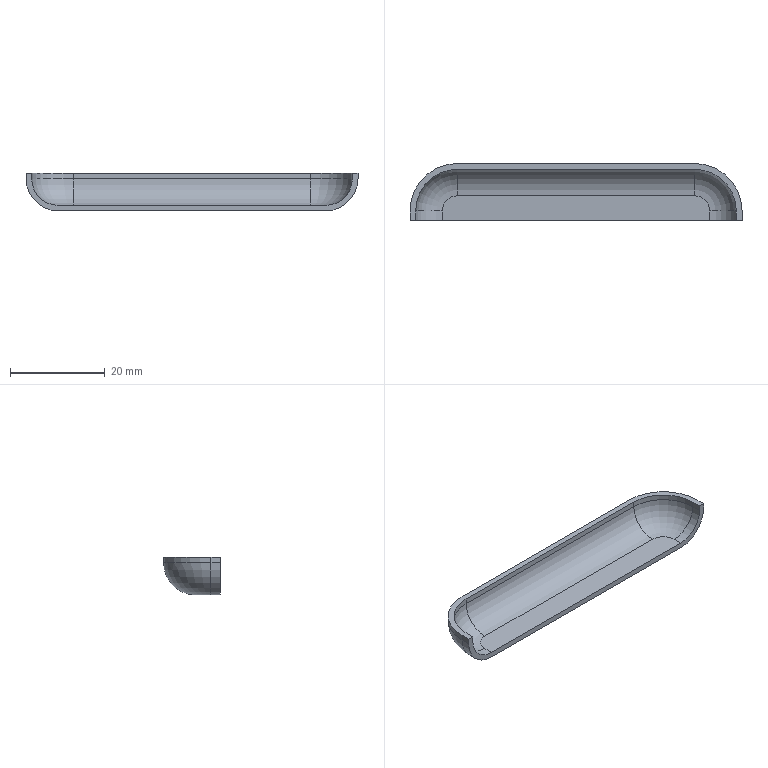Component | SolidWorks | LeftDoorPanelAssembly-1_LeftDoorPanelWeldment-1_LouverSupplement-12 | 1 solid | 24 faces | box 70 x 12 x 8 mm | volume 1361 mm3 | cylinder 10 | plane 10 | torus 4 | commonest cylinder face diameters 13.6 x3 11.2 x3 20 x2 17.6 x2
build123d program:
from build123d import *

# Parameters (mm, degrees)
BOSS_EXTRUDE1_DEPTH = 8
FILLET1_R           = 6.8
SHELL1_T            = -1.2


with BuildPart() as part:
    # Sketch1 → Boss-Extrude1 (new body)
    with BuildSketch(Plane.XY):
        with BuildLine():
            Line((-25, 12), (25, 12))
            ThreePointArc((25, 12), (32.071, 9.071), (35, 2))
            Line((35, 2), (35, 0))
            Line((35, 0), (-35, 0))
            Line((-35, 0), (-35, 2))
            ThreePointArc((-35, 2), (-32.071, 9.071), (-25, 12))
        make_face()
    extrude(amount=BOSS_EXTRUDE1_DEPTH)

    # Fillet1
    fillet1_edges = [part.edges().sort_by_distance(p)[0] for p in [
        (35, 1, 8),
        (32.071, 9.071, 8),
        (0, 12, 8),
        (-32.071, 9.071, 8),
        (-35, 1, 8),
    ]]
    fillet(fillet1_edges, radius=FILLET1_R)

    # Shell1
    shell1_openings = [part.faces().sort_by_distance(p)[0] for p in [
        (0, 0, 3.909),
        (0, 5.797, 0),
    ]]
    offset(amount=SHELL1_T, openings=shell1_openings, kind=Kind.INTERSECTION)


solid = part.part

# Placed as in the assembly
solid = solid.moved(Location((224.337, 24.042, -71.9), (-180, 0, 180)))
STEP:
#1=COLOUR_RGB('',0.7922,0.8196,0.9333);
#2=FILL_AREA_STYLE_COLOUR('',#1);
#3=FILL_AREA_STYLE('',(#2));
#4=SURFACE_STYLE_FILL_AREA(#3);
#5=SURFACE_SIDE_STYLE('',(#4));
#6=SURFACE_STYLE_USAGE(.BOTH.,#5);
#7=PRESENTATION_STYLE_ASSIGNMENT((#6));
#8=CARTESIAN_POINT('',(10.21,1.025,-2.878));
#9=VERTEX_POINT('',#8);
#10=CARTESIAN_POINT('',(10.21,1.025,-2.831));
#11=VERTEX_POINT('',#10);
#12=CARTESIAN_POINT('',(10.21,1.025,-3.146));
#13=DIRECTION('',(-0.,0.,1.));
#14=VECTOR('',#13,39.37);
#15=LINE('',#12,#14);
#16=EDGE_CURVE('',#9,#11,#15,.T.);
#17=ORIENTED_EDGE('',*,*,#16,.F.);
#18=CARTESIAN_POINT('',(9.816,1.419,-2.878));
#19=VERTEX_POINT('',#18);
#20=CARTESIAN_POINT('',(9.816,1.025,-2.878));
#21=DIRECTION('',(-0.,0.,1.));
#22=DIRECTION('',(-1.,-0.,-0.));
#23=AXIS2_PLACEMENT_3D('',#20,#21,#22);
#24=CIRCLE('',#23,0.3937);
#25=EDGE_CURVE('',#9,#19,#24,.T.);
#26=ORIENTED_EDGE('',*,*,#25,.T.);
#27=CARTESIAN_POINT('',(9.816,1.419,-2.831));
#28=VERTEX_POINT('',#27);
#29=CARTESIAN_POINT('',(9.816,1.419,-3.146));
#30=DIRECTION('',(-0.,0.,1.));
#31=VECTOR('',#30,39.37);
#32=LINE('',#29,#31);
#33=EDGE_CURVE('',#19,#28,#32,.T.);
#34=ORIENTED_EDGE('',*,*,#33,.T.);
#35=CARTESIAN_POINT('',(9.816,1.025,-2.831));
#36=DIRECTION('',(0.,-0.,-1.));
#37=DIRECTION('',(-1.,-0.,-0.));
#38=AXIS2_PLACEMENT_3D('',#35,#36,#37);
#39=CIRCLE('',#38,0.3937);
#40=EDGE_CURVE('',#28,#11,#39,.T.);
#41=ORIENTED_EDGE('',*,*,#40,.T.);
#42=EDGE_LOOP('',(#17,#26,#34,#41));
#43=FACE_OUTER_BOUND('',#42,.T.);
#44=CARTESIAN_POINT('',(9.816,1.025,-3.146));
#45=DIRECTION('',(-0.,0.,1.));
#46=DIRECTION('',(1.,0.,0.));
#47=AXIS2_PLACEMENT_3D('',#44,#45,#46);
#48=CYLINDRICAL_SURFACE('',#47,0.3937);
#49=ADVANCED_FACE('',(#43),#48,.T.);
#50=CARTESIAN_POINT('',(10.21,0.9465,-2.878));
#51=VERTEX_POINT('',#50);
#52=CARTESIAN_POINT('',(10.21,0.9465,-2.831));
#53=VERTEX_POINT('',#52);
#54=CARTESIAN_POINT('',(10.21,0.9465,-3.146));
#55=DIRECTION('',(-0.,0.,1.));
#56=VECTOR('',#55,39.37);
#57=LINE('',#54,#56);
#58=EDGE_CURVE('',#51,#53,#57,.T.);
#59=ORIENTED_EDGE('',*,*,#58,.F.);
#60=CARTESIAN_POINT('',(10.21,1.025,-2.878));
#61=DIRECTION('',(-0.,1.,-0.));
#62=VECTOR('',#61,39.37);
#63=LINE('',#60,#62);
#64=EDGE_CURVE('',#51,#9,#63,.T.);
#65=ORIENTED_EDGE('',*,*,#64,.T.);
#66=ORIENTED_EDGE('',*,*,#16,.T.);
#67=CARTESIAN_POINT('',(10.21,0.9465,-2.831));
#68=DIRECTION('',(0.,-1.,0.));
#69=VECTOR('',#68,39.37);
#70=LINE('',#67,#69);
#71=EDGE_CURVE('',#11,#53,#70,.T.);
#72=ORIENTED_EDGE('',*,*,#71,.T.);
#73=EDGE_LOOP('',(#59,#65,#66,#72));
#74=FACE_OUTER_BOUND('',#73,.T.);
#75=CARTESIAN_POINT('',(10.21,0.9465,-3.146));
#76=DIRECTION('',(-1.,-0.,-0.));
#77=DIRECTION('',(-0.,0.,1.));
#78=AXIS2_PLACEMENT_3D('',#75,#76,#77);
#79=PLANE('',#78);
#80=ADVANCED_FACE('',(#74),#79,.F.);
#81=CARTESIAN_POINT('',(7.501,0.9465,-2.878));
#82=VERTEX_POINT('',#81);
#83=CARTESIAN_POINT('',(7.722,0.9465,-3.098));
#84=VERTEX_POINT('',#83);
#85=CARTESIAN_POINT('',(7.722,0.9465,-2.878));
#86=DIRECTION('',(0.,-1.,0.));
#87=DIRECTION('',(0.,-0.,-1.));
#88=AXIS2_PLACEMENT_3D('',#85,#86,#87);
#89=CIRCLE('',#88,0.2205);
#90=EDGE_CURVE('',#82,#84,#89,.T.);
#91=ORIENTED_EDGE('',*,*,#90,.F.);
#92=CARTESIAN_POINT('',(7.501,0.9465,-2.831));
#93=VERTEX_POINT('',#92);
#94=CARTESIAN_POINT('',(7.501,0.9465,-3.146));
#95=DIRECTION('',(-0.,0.,1.));
#96=VECTOR('',#95,39.37);
#97=LINE('',#94,#96);
#98=EDGE_CURVE('',#82,#93,#97,.T.);
#99=ORIENTED_EDGE('',*,*,#98,.T.);
#100=CARTESIAN_POINT('',(7.454,0.9465,-2.831));
#101=VERTEX_POINT('',#100);
#102=CARTESIAN_POINT('',(10.21,0.9465,-2.831));
#103=DIRECTION('',(-1.,-0.,-0.));
#104=VECTOR('',#103,39.37);
#105=LINE('',#102,#104);
#106=EDGE_CURVE('',#93,#101,#105,.T.);
#107=ORIENTED_EDGE('',*,*,#106,.T.);
#108=CARTESIAN_POINT('',(7.454,0.9465,-2.878));
#109=VERTEX_POINT('',#108);
#110=CARTESIAN_POINT('',(7.454,0.9465,-3.146));
#111=DIRECTION('',(-0.,0.,1.));
#112=VECTOR('',#111,39.37);
#113=LINE('',#110,#112);
#114=EDGE_CURVE('',#109,#101,#113,.T.);
#115=ORIENTED_EDGE('',*,*,#114,.F.);
#116=CARTESIAN_POINT('',(7.722,0.9465,-3.146));
#117=VERTEX_POINT('',#116);
#118=CARTESIAN_POINT('',(7.722,0.9465,-2.878));
#119=DIRECTION('',(0.,-1.,0.));
#120=DIRECTION('',(0.,-0.,-1.));
#121=AXIS2_PLACEMENT_3D('',#118,#119,#120);
#122=CIRCLE('',#121,0.2677);
#123=EDGE_CURVE('',#109,#117,#122,.T.);
#124=ORIENTED_EDGE('',*,*,#123,.T.);
#125=CARTESIAN_POINT('',(9.942,0.9465,-3.146));
#126=VERTEX_POINT('',#125);
#127=CARTESIAN_POINT('',(10.21,0.9465,-3.146));
#128=DIRECTION('',(-1.,-0.,-0.));
#129=VECTOR('',#128,39.37);
#130=LINE('',#127,#129);
#131=EDGE_CURVE('',#126,#117,#130,.T.);
#132=ORIENTED_EDGE('',*,*,#131,.F.);
#133=CARTESIAN_POINT('',(9.942,0.9465,-2.878));
#134=DIRECTION('',(0.,-1.,0.));
#135=DIRECTION('',(0.,-0.,-1.));
#136=AXIS2_PLACEMENT_3D('',#133,#134,#135);
#137=CIRCLE('',#136,0.2677);
#138=EDGE_CURVE('',#126,#51,#137,.T.);
#139=ORIENTED_EDGE('',*,*,#138,.T.);
#140=ORIENTED_EDGE('',*,*,#58,.T.);
#141=CARTESIAN_POINT('',(10.163,0.9465,-2.831));
#142=VERTEX_POINT('',#141);
#143=CARTESIAN_POINT('',(10.21,0.9465,-2.831));
#144=DIRECTION('',(-1.,-0.,-0.));
#145=VECTOR('',#144,39.37);
#146=LINE('',#143,#145);
#147=EDGE_CURVE('',#53,#142,#146,.T.);
#148=ORIENTED_EDGE('',*,*,#147,.T.);
#149=CARTESIAN_POINT('',(10.163,0.9465,-2.878));
#150=VERTEX_POINT('',#149);
#151=CARTESIAN_POINT('',(10.163,0.9465,-3.146));
#152=DIRECTION('',(-0.,0.,1.));
#153=VECTOR('',#152,39.37);
#154=LINE('',#151,#153);
#155=EDGE_CURVE('',#150,#142,#154,.T.);
#156=ORIENTED_EDGE('',*,*,#155,.F.);
#157=CARTESIAN_POINT('',(9.942,0.9465,-3.098));
#158=VERTEX_POINT('',#157);
#159=CARTESIAN_POINT('',(9.942,0.9465,-2.878));
#160=DIRECTION('',(0.,-1.,0.));
#161=DIRECTION('',(0.,-0.,-1.));
#162=AXIS2_PLACEMENT_3D('',#159,#160,#161);
#163=CIRCLE('',#162,0.2205);
#164=EDGE_CURVE('',#158,#150,#163,.T.);
#165=ORIENTED_EDGE('',*,*,#164,.F.);
#166=CARTESIAN_POINT('',(10.21,0.9465,-3.098));
#167=DIRECTION('',(-1.,-0.,-0.));
#168=VECTOR('',#167,39.37);
#169=LINE('',#166,#168);
#170=EDGE_CURVE('',#158,#84,#169,.T.);
#171=ORIENTED_EDGE('',*,*,#170,.T.);
#172=EDGE_LOOP('',(#91,#99,#107,#115,#124,#132,#139,#140,#148,#156,#165,#171));
#173=FACE_OUTER_BOUND('',#172,.T.);
#174=CARTESIAN_POINT('',(10.21,0.9465,-3.146));
#175=DIRECTION('',(-0.,1.,-0.));
#176=DIRECTION('',(0.,-0.,-1.));
#177=AXIS2_PLACEMENT_3D('',#174,#175,#176);
#178=PLANE('',#177);
#179=ADVANCED_FACE('',(#173),#178,.F.);
#180=CARTESIAN_POINT('',(7.454,1.025,-2.878));
#181=VERTEX_POINT('',#180);
#182=CARTESIAN_POINT('',(7.454,1.025,-2.831));
#183=VERTEX_POINT('',#182);
#184=CARTESIAN_POINT('',(7.454,1.025,-3.146));
#185=DIRECTION('',(-0.,0.,1.));
#186=VECTOR('',#185,39.37);
#187=LINE('',#184,#186);
#188=EDGE_CURVE('',#181,#183,#187,.T.);
#189=ORIENTED_EDGE('',*,*,#188,.F.);
#190=CARTESIAN_POINT('',(7.454,0.9465,-2.878));
#191=DIRECTION('',(0.,-1.,0.));
#192=VECTOR('',#191,39.37);
#193=LINE('',#190,#192);
#194=EDGE_CURVE('',#181,#109,#193,.T.);
#195=ORIENTED_EDGE('',*,*,#194,.T.);
#196=ORIENTED_EDGE('',*,*,#114,.T.);
#197=CARTESIAN_POINT('',(7.454,0.9465,-2.831));
#198=DIRECTION('',(-0.,1.,-0.));
#199=VECTOR('',#198,39.37);
#200=LINE('',#197,#199);
#201=EDGE_CURVE('',#101,#183,#200,.T.);
#202=ORIENTED_EDGE('',*,*,#201,.T.);
#203=EDGE_LOOP('',(#189,#195,#196,#202));
#204=FACE_OUTER_BOUND('',#203,.T.);
#205=CARTESIAN_POINT('',(7.454,0.9465,-3.146));
#206=DIRECTION('',(1.,0.,0.));
#207=DIRECTION('',(0.,-0.,-1.));
#208=AXIS2_PLACEMENT_3D('',#205,#206,#207);
#209=PLANE('',#208);
#210=ADVANCED_FACE('',(#204),#209,.F.);
#211=CARTESIAN_POINT('',(7.848,1.419,-2.878));
#212=VERTEX_POINT('',#211);
#213=CARTESIAN_POINT('',(7.848,1.419,-2.831));
#214=VERTEX_POINT('',#213);
#215=CARTESIAN_POINT('',(7.848,1.419,-3.146));
#216=DIRECTION('',(-0.,0.,1.));
#217=VECTOR('',#216,39.37);
#218=LINE('',#215,#217);
#219=EDGE_CURVE('',#212,#214,#218,.T.);
#220=ORIENTED_EDGE('',*,*,#219,.F.);
#221=CARTESIAN_POINT('',(7.848,1.025,-2.878));
#222=DIRECTION('',(-0.,0.,1.));
#223=DIRECTION('',(-1.,-0.,-0.));
#224=AXIS2_PLACEMENT_3D('',#221,#222,#223);
#225=CIRCLE('',#224,0.3937);
#226=EDGE_CURVE('',#212,#181,#225,.T.);
#227=ORIENTED_EDGE('',*,*,#226,.T.);
#228=ORIENTED_EDGE('',*,*,#188,.T.);
#229=CARTESIAN_POINT('',(7.848,1.025,-2.831));
#230=DIRECTION('',(0.,-0.,-1.));
#231=DIRECTION('',(-1.,-0.,-0.));
#232=AXIS2_PLACEMENT_3D('',#229,#230,#231);
#233=CIRCLE('',#232,0.3937);
#234=EDGE_CURVE('',#183,#214,#233,.T.);
#235=ORIENTED_EDGE('',*,*,#234,.T.);
#236=EDGE_LOOP('',(#220,#227,#228,#235));
#237=FACE_OUTER_BOUND('',#236,.T.);
#238=CARTESIAN_POINT('',(7.848,1.025,-3.146));
#239=DIRECTION('',(-0.,0.,1.));
#240=DIRECTION('',(1.,0.,0.));
#241=AXIS2_PLACEMENT_3D('',#238,#239,#240);
#242=CYLINDRICAL_SURFACE('',#241,0.3937);
#243=ADVANCED_FACE('',(#237),#242,.T.);
#244=ORIENTED_EDGE('',*,*,#33,.F.);
#245=CARTESIAN_POINT('',(7.848,1.419,-2.878));
#246=DIRECTION('',(-1.,-0.,-0.));
#247=VECTOR('',#246,39.37);
#248=LINE('',#245,#247);
#249=EDGE_CURVE('',#19,#212,#248,.T.);
#250=ORIENTED_EDGE('',*,*,#249,.T.);
#251=ORIENTED_EDGE('',*,*,#219,.T.);
#252=CARTESIAN_POINT('',(9.816,1.419,-2.831));
#253=DIRECTION('',(1.,0.,0.));
#254=VECTOR('',#253,39.37);
#255=LINE('',#252,#254);
#256=EDGE_CURVE('',#214,#28,#255,.T.);
#257=ORIENTED_EDGE('',*,*,#256,.T.);
#258=EDGE_LOOP('',(#244,#250,#251,#257));
#259=FACE_OUTER_BOUND('',#258,.T.);
#260=CARTESIAN_POINT('',(9.816,1.419,-3.146));
#261=DIRECTION('',(0.,-1.,0.));
#262=DIRECTION('',(-0.,0.,1.));
#263=AXIS2_PLACEMENT_3D('',#260,#261,#262);
#264=PLANE('',#263);
#265=ADVANCED_FACE('',(#259),#264,.F.);
#266=ORIENTED_EDGE('',*,*,#131,.T.);
#267=CARTESIAN_POINT('',(7.722,1.025,-3.146));
#268=VERTEX_POINT('',#267);
#269=CARTESIAN_POINT('',(7.722,1.025,-3.146));
#270=DIRECTION('',(-0.,1.,-0.));
#271=VECTOR('',#270,39.37);
#272=LINE('',#269,#271);
#273=EDGE_CURVE('',#117,#268,#272,.T.);
#274=ORIENTED_EDGE('',*,*,#273,.T.);
#275=CARTESIAN_POINT('',(7.848,1.151,-3.146));
#276=VERTEX_POINT('',#275);
#277=CARTESIAN_POINT('',(7.848,1.025,-3.146));
#278=DIRECTION('',(0.,-0.,-1.));
#279=DIRECTION('',(-1.,-0.,-0.));
#280=AXIS2_PLACEMENT_3D('',#277,#278,#279);
#281=CIRCLE('',#280,0.126);
#282=EDGE_CURVE('',#268,#276,#281,.T.);
#283=ORIENTED_EDGE('',*,*,#282,.T.);
#284=CARTESIAN_POINT('',(9.816,1.151,-3.146));
#285=VERTEX_POINT('',#284);
#286=CARTESIAN_POINT('',(9.816,1.151,-3.146));
#287=DIRECTION('',(1.,0.,0.));
#288=VECTOR('',#287,39.37);
#289=LINE('',#286,#288);
#290=EDGE_CURVE('',#276,#285,#289,.T.);
#291=ORIENTED_EDGE('',*,*,#290,.T.);
#292=CARTESIAN_POINT('',(9.942,1.025,-3.146));
#293=VERTEX_POINT('',#292);
#294=CARTESIAN_POINT('',(9.816,1.025,-3.146));
#295=DIRECTION('',(0.,-0.,-1.));
#296=DIRECTION('',(-1.,-0.,-0.));
#297=AXIS2_PLACEMENT_3D('',#294,#295,#296);
#298=CIRCLE('',#297,0.126);
#299=EDGE_CURVE('',#285,#293,#298,.T.);
#300=ORIENTED_EDGE('',*,*,#299,.T.);
#301=CARTESIAN_POINT('',(9.942,0.9465,-3.146));
#302=DIRECTION('',(0.,-1.,0.));
#303=VECTOR('',#302,39.37);
#304=LINE('',#301,#303);
#305=EDGE_CURVE('',#293,#126,#304,.T.);
#306=ORIENTED_EDGE('',*,*,#305,.T.);
#307=EDGE_LOOP('',(#266,#274,#283,#291,#300,#306));
#308=FACE_OUTER_BOUND('',#307,.T.);
#309=CARTESIAN_POINT('',(9.816,1.025,-3.146));
#310=DIRECTION('',(0.,-0.,-1.));
#311=DIRECTION('',(-1.,-0.,-0.));
#312=AXIS2_PLACEMENT_3D('',#309,#310,#311);
#313=PLANE('',#312);
#314=ADVANCED_FACE('',(#308),#313,.T.);
#315=ORIENTED_EDGE('',*,*,#106,.F.);
#316=CARTESIAN_POINT('',(7.501,1.025,-2.831));
#317=VERTEX_POINT('',#316);
#318=CARTESIAN_POINT('',(7.501,0.9465,-2.831));
#319=DIRECTION('',(-0.,1.,-0.));
#320=VECTOR('',#319,39.37);
#321=LINE('',#318,#320);
#322=EDGE_CURVE('',#93,#317,#321,.T.);
#323=ORIENTED_EDGE('',*,*,#322,.T.);
#324=CARTESIAN_POINT('',(7.848,1.372,-2.831));
#325=VERTEX_POINT('',#324);
#326=CARTESIAN_POINT('',(7.848,1.025,-2.831));
#327=DIRECTION('',(0.,-0.,-1.));
#328=DIRECTION('',(-1.,-0.,-0.));
#329=AXIS2_PLACEMENT_3D('',#326,#327,#328);
#330=CIRCLE('',#329,0.3465);
#331=EDGE_CURVE('',#317,#325,#330,.T.);
#332=ORIENTED_EDGE('',*,*,#331,.T.);
#333=CARTESIAN_POINT('',(9.816,1.372,-2.831));
#334=VERTEX_POINT('',#333);
#335=CARTESIAN_POINT('',(9.816,1.372,-2.831));
#336=DIRECTION('',(1.,0.,0.));
#337=VECTOR('',#336,39.37);
#338=LINE('',#335,#337);
#339=EDGE_CURVE('',#325,#334,#338,.T.);
#340=ORIENTED_EDGE('',*,*,#339,.T.);
#341=CARTESIAN_POINT('',(10.163,1.025,-2.831));
#342=VERTEX_POINT('',#341);
#343=CARTESIAN_POINT('',(9.816,1.025,-2.831));
#344=DIRECTION('',(0.,-0.,-1.));
#345=DIRECTION('',(-1.,-0.,-0.));
#346=AXIS2_PLACEMENT_3D('',#343,#344,#345);
#347=CIRCLE('',#346,0.3465);
#348=EDGE_CURVE('',#334,#342,#347,.T.);
#349=ORIENTED_EDGE('',*,*,#348,.T.);
#350=CARTESIAN_POINT('',(10.163,0.9465,-2.831));
#351=DIRECTION('',(0.,-1.,0.));
#352=VECTOR('',#351,39.37);
#353=LINE('',#350,#352);
#354=EDGE_CURVE('',#342,#142,#353,.T.);
#355=ORIENTED_EDGE('',*,*,#354,.T.);
#356=ORIENTED_EDGE('',*,*,#147,.F.);
#357=ORIENTED_EDGE('',*,*,#71,.F.);
#358=ORIENTED_EDGE('',*,*,#40,.F.);
#359=ORIENTED_EDGE('',*,*,#256,.F.);
#360=ORIENTED_EDGE('',*,*,#234,.F.);
#361=ORIENTED_EDGE('',*,*,#201,.F.);
#362=EDGE_LOOP('',(#315,#323,#332,#340,#349,#355,#356,#357,#358,#359,#360,#361));
#363=FACE_OUTER_BOUND('',#362,.T.);
#364=CARTESIAN_POINT('',(9.816,1.025,-2.831));
#365=DIRECTION('',(0.,-0.,-1.));
#366=DIRECTION('',(-1.,-0.,-0.));
#367=AXIS2_PLACEMENT_3D('',#364,#365,#366);
#368=PLANE('',#367);
#369=ADVANCED_FACE('',(#363),#368,.F.);
#370=ORIENTED_EDGE('',*,*,#138,.F.);
#371=ORIENTED_EDGE('',*,*,#305,.F.);
#372=CARTESIAN_POINT('',(9.942,1.025,-2.878));
#373=DIRECTION('',(-0.,1.,-0.));
#374=DIRECTION('',(0.,-0.,-1.));
#375=AXIS2_PLACEMENT_3D('',#372,#373,#374);
#376=CIRCLE('',#375,0.2677);
#377=EDGE_CURVE('',#9,#293,#376,.T.);
#378=ORIENTED_EDGE('',*,*,#377,.F.);
#379=ORIENTED_EDGE('',*,*,#64,.F.);
#380=EDGE_LOOP('',(#370,#371,#378,#379));
#381=FACE_OUTER_BOUND('',#380,.T.);
#382=CARTESIAN_POINT('',(9.942,1.025,-2.878));
#383=DIRECTION('',(-0.,1.,-0.));
#384=DIRECTION('',(0.,-0.,-1.));
#385=AXIS2_PLACEMENT_3D('',#382,#383,#384);
#386=CYLINDRICAL_SURFACE('',#385,0.2677);
#387=ADVANCED_FACE('',(#381),#386,.T.);
#388=ORIENTED_EDGE('',*,*,#377,.T.);
#389=ORIENTED_EDGE('',*,*,#299,.F.);
#390=CARTESIAN_POINT('',(9.816,1.151,-2.878));
#391=DIRECTION('',(-1.,-0.,-0.));
#392=DIRECTION('',(-0.,0.,1.));
#393=AXIS2_PLACEMENT_3D('',#390,#391,#392);
#394=CIRCLE('',#393,0.2677);
#395=EDGE_CURVE('',#19,#285,#394,.T.);
#396=ORIENTED_EDGE('',*,*,#395,.F.);
#397=ORIENTED_EDGE('',*,*,#25,.F.);
#398=EDGE_LOOP('',(#388,#389,#396,#397));
#399=FACE_OUTER_BOUND('',#398,.T.);
#400=CARTESIAN_POINT('',(9.816,1.025,-2.878));
#401=DIRECTION('',(0.,-0.,-1.));
#402=DIRECTION('',(-1.,-0.,-0.));
#403=AXIS2_PLACEMENT_3D('',#400,#401,#402);
#404=TOROIDAL_SURFACE('',#403,0.126,0.2677);
#405=ADVANCED_FACE('',(#399),#404,.T.);
#406=ORIENTED_EDGE('',*,*,#395,.T.);
#407=ORIENTED_EDGE('',*,*,#290,.F.);
#408=CARTESIAN_POINT('',(7.848,1.151,-2.878));
#409=DIRECTION('',(-1.,-0.,-0.));
#410=DIRECTION('',(-0.,0.,1.));
#411=AXIS2_PLACEMENT_3D('',#408,#409,#410);
#412=CIRCLE('',#411,0.2677);
#413=EDGE_CURVE('',#212,#276,#412,.T.);
#414=ORIENTED_EDGE('',*,*,#413,.F.);
#415=ORIENTED_EDGE('',*,*,#249,.F.);
#416=EDGE_LOOP('',(#406,#407,#414,#415));
#417=FACE_OUTER_BOUND('',#416,.T.);
#418=CARTESIAN_POINT('',(9.816,1.151,-2.878));
#419=DIRECTION('',(-1.,-0.,-0.));
#420=DIRECTION('',(-0.,0.,1.));
#421=AXIS2_PLACEMENT_3D('',#418,#419,#420);
#422=CYLINDRICAL_SURFACE('',#421,0.2677);
#423=ADVANCED_FACE('',(#417),#422,.T.);
#424=ORIENTED_EDGE('',*,*,#413,.T.);
#425=ORIENTED_EDGE('',*,*,#282,.F.);
#426=CARTESIAN_POINT('',(7.722,1.025,-2.878));
#427=DIRECTION('',(0.,-1.,0.));
#428=DIRECTION('',(-0.,0.,1.));
#429=AXIS2_PLACEMENT_3D('',#426,#427,#428);
#430=CIRCLE('',#429,0.2677);
#431=EDGE_CURVE('',#181,#268,#430,.T.);
#432=ORIENTED_EDGE('',*,*,#431,.F.);
#433=ORIENTED_EDGE('',*,*,#226,.F.);
#434=EDGE_LOOP('',(#424,#425,#432,#433));
#435=FACE_OUTER_BOUND('',#434,.T.);
#436=CARTESIAN_POINT('',(7.848,1.025,-2.878));
#437=DIRECTION('',(0.,-0.,-1.));
#438=DIRECTION('',(-1.,-0.,-0.));
#439=AXIS2_PLACEMENT_3D('',#436,#437,#438);
#440=TOROIDAL_SURFACE('',#439,0.126,0.2677);
#441=ADVANCED_FACE('',(#435),#440,.T.);
#442=ORIENTED_EDGE('',*,*,#123,.F.);
#443=ORIENTED_EDGE('',*,*,#194,.F.);
#444=ORIENTED_EDGE('',*,*,#431,.T.);
#445=ORIENTED_EDGE('',*,*,#273,.F.);
#446=EDGE_LOOP('',(#442,#443,#444,#445));
#447=FACE_OUTER_BOUND('',#446,.T.);
#448=CARTESIAN_POINT('',(7.722,1.025,-2.878));
#449=DIRECTION('',(0.,-1.,0.));
#450=DIRECTION('',(-0.,0.,1.));
#451=AXIS2_PLACEMENT_3D('',#448,#449,#450);
#452=CYLINDRICAL_SURFACE('',#451,0.2677);
#453=ADVANCED_FACE('',(#447),#452,.T.);
#454=CARTESIAN_POINT('',(10.163,1.025,-2.878));
#455=VERTEX_POINT('',#454);
#456=CARTESIAN_POINT('',(10.163,1.025,-3.146));
#457=DIRECTION('',(-0.,0.,1.));
#458=VECTOR('',#457,39.37);
#459=LINE('',#456,#458);
#460=EDGE_CURVE('',#455,#342,#459,.T.);
#461=ORIENTED_EDGE('',*,*,#460,.T.);
#462=ORIENTED_EDGE('',*,*,#348,.F.);
#463=CARTESIAN_POINT('',(9.816,1.372,-2.878));
#464=VERTEX_POINT('',#463);
#465=CARTESIAN_POINT('',(9.816,1.372,-3.146));
#466=DIRECTION('',(-0.,0.,1.));
#467=VECTOR('',#466,39.37);
#468=LINE('',#465,#467);
#469=EDGE_CURVE('',#464,#334,#468,.T.);
#470=ORIENTED_EDGE('',*,*,#469,.F.);
#471=CARTESIAN_POINT('',(9.816,1.025,-2.878));
#472=DIRECTION('',(-0.,0.,1.));
#473=DIRECTION('',(1.,0.,0.));
#474=AXIS2_PLACEMENT_3D('',#471,#472,#473);
#475=CIRCLE('',#474,0.3465);
#476=EDGE_CURVE('',#455,#464,#475,.T.);
#477=ORIENTED_EDGE('',*,*,#476,.F.);
#478=EDGE_LOOP('',(#461,#462,#470,#477));
#479=FACE_OUTER_BOUND('',#478,.T.);
#480=CARTESIAN_POINT('',(9.816,1.025,-3.146));
#481=DIRECTION('',(-0.,0.,1.));
#482=DIRECTION('',(1.,0.,0.));
#483=AXIS2_PLACEMENT_3D('',#480,#481,#482);
#484=CYLINDRICAL_SURFACE('',#483,0.3465);
#485=ADVANCED_FACE('',(#479),#484,.F.);
#486=ORIENTED_EDGE('',*,*,#155,.T.);
#487=ORIENTED_EDGE('',*,*,#354,.F.);
#488=ORIENTED_EDGE('',*,*,#460,.F.);
#489=CARTESIAN_POINT('',(10.163,0.9465,-2.878));
#490=DIRECTION('',(-0.,1.,-0.));
#491=VECTOR('',#490,39.37);
#492=LINE('',#489,#491);
#493=EDGE_CURVE('',#150,#455,#492,.T.);
#494=ORIENTED_EDGE('',*,*,#493,.F.);
#495=EDGE_LOOP('',(#486,#487,#488,#494));
#496=FACE_OUTER_BOUND('',#495,.T.);
#497=CARTESIAN_POINT('',(10.163,0.9465,-3.146));
#498=DIRECTION('',(-1.,-0.,-0.));
#499=DIRECTION('',(-0.,0.,1.));
#500=AXIS2_PLACEMENT_3D('',#497,#498,#499);
#501=PLANE('',#500);
#502=ADVANCED_FACE('',(#496),#501,.T.);
#503=CARTESIAN_POINT('',(7.501,1.025,-2.878));
#504=VERTEX_POINT('',#503);
#505=CARTESIAN_POINT('',(7.501,1.025,-3.146));
#506=DIRECTION('',(-0.,0.,1.));
#507=VECTOR('',#506,39.37);
#508=LINE('',#505,#507);
#509=EDGE_CURVE('',#504,#317,#508,.T.);
#510=ORIENTED_EDGE('',*,*,#509,.T.);
#511=ORIENTED_EDGE('',*,*,#322,.F.);
#512=ORIENTED_EDGE('',*,*,#98,.F.);
#513=CARTESIAN_POINT('',(7.501,0.9465,-2.878));
#514=DIRECTION('',(0.,-1.,0.));
#515=VECTOR('',#514,39.37);
#516=LINE('',#513,#515);
#517=EDGE_CURVE('',#504,#82,#516,.T.);
#518=ORIENTED_EDGE('',*,*,#517,.F.);
#519=EDGE_LOOP('',(#510,#511,#512,#518));
#520=FACE_OUTER_BOUND('',#519,.T.);
#521=CARTESIAN_POINT('',(7.501,0.9465,-3.146));
#522=DIRECTION('',(1.,0.,0.));
#523=DIRECTION('',(0.,-0.,-1.));
#524=AXIS2_PLACEMENT_3D('',#521,#522,#523);
#525=PLANE('',#524);
#526=ADVANCED_FACE('',(#520),#525,.T.);
#527=CARTESIAN_POINT('',(7.848,1.372,-2.878));
#528=VERTEX_POINT('',#527);
#529=CARTESIAN_POINT('',(7.848,1.372,-3.146));
#530=DIRECTION('',(-0.,0.,1.));
#531=VECTOR('',#530,39.37);
#532=LINE('',#529,#531);
#533=EDGE_CURVE('',#528,#325,#532,.T.);
#534=ORIENTED_EDGE('',*,*,#533,.T.);
#535=ORIENTED_EDGE('',*,*,#331,.F.);
#536=ORIENTED_EDGE('',*,*,#509,.F.);
#537=CARTESIAN_POINT('',(7.848,1.025,-2.878));
#538=DIRECTION('',(-0.,0.,1.));
#539=DIRECTION('',(1.,0.,0.));
#540=AXIS2_PLACEMENT_3D('',#537,#538,#539);
#541=CIRCLE('',#540,0.3465);
#542=EDGE_CURVE('',#528,#504,#541,.T.);
#543=ORIENTED_EDGE('',*,*,#542,.F.);
#544=EDGE_LOOP('',(#534,#535,#536,#543));
#545=FACE_OUTER_BOUND('',#544,.T.);
#546=CARTESIAN_POINT('',(7.848,1.025,-3.146));
#547=DIRECTION('',(-0.,0.,1.));
#548=DIRECTION('',(1.,0.,0.));
#549=AXIS2_PLACEMENT_3D('',#546,#547,#548);
#550=CYLINDRICAL_SURFACE('',#549,0.3465);
#551=ADVANCED_FACE('',(#545),#550,.F.);
#552=ORIENTED_EDGE('',*,*,#469,.T.);
#553=ORIENTED_EDGE('',*,*,#339,.F.);
#554=ORIENTED_EDGE('',*,*,#533,.F.);
#555=CARTESIAN_POINT('',(9.816,1.372,-2.878));
#556=DIRECTION('',(-1.,-0.,-0.));
#557=VECTOR('',#556,39.37);
#558=LINE('',#555,#557);
#559=EDGE_CURVE('',#464,#528,#558,.T.);
#560=ORIENTED_EDGE('',*,*,#559,.F.);
#561=EDGE_LOOP('',(#552,#553,#554,#560));
#562=FACE_OUTER_BOUND('',#561,.T.);
#563=CARTESIAN_POINT('',(9.816,1.372,-3.146));
#564=DIRECTION('',(0.,-1.,0.));
#565=DIRECTION('',(-0.,0.,1.));
#566=AXIS2_PLACEMENT_3D('',#563,#564,#565);
#567=PLANE('',#566);
#568=ADVANCED_FACE('',(#562),#567,.T.);
#569=ORIENTED_EDGE('',*,*,#170,.F.);
#570=CARTESIAN_POINT('',(9.942,1.025,-3.098));
#571=VERTEX_POINT('',#570);
#572=CARTESIAN_POINT('',(9.942,1.025,-3.098));
#573=DIRECTION('',(0.,-1.,0.));
#574=VECTOR('',#573,39.37);
#575=LINE('',#572,#574);
#576=EDGE_CURVE('',#571,#158,#575,.T.);
#577=ORIENTED_EDGE('',*,*,#576,.F.);
#578=CARTESIAN_POINT('',(9.816,1.151,-3.098));
#579=VERTEX_POINT('',#578);
#580=CARTESIAN_POINT('',(9.816,1.025,-3.098));
#581=DIRECTION('',(0.,-0.,-1.));
#582=DIRECTION('',(-1.,-0.,-0.));
#583=AXIS2_PLACEMENT_3D('',#580,#581,#582);
#584=CIRCLE('',#583,0.126);
#585=EDGE_CURVE('',#579,#571,#584,.T.);
#586=ORIENTED_EDGE('',*,*,#585,.F.);
#587=CARTESIAN_POINT('',(7.848,1.151,-3.098));
#588=VERTEX_POINT('',#587);
#589=CARTESIAN_POINT('',(9.816,1.151,-3.098));
#590=DIRECTION('',(1.,0.,0.));
#591=VECTOR('',#590,39.37);
#592=LINE('',#589,#591);
#593=EDGE_CURVE('',#588,#579,#592,.T.);
#594=ORIENTED_EDGE('',*,*,#593,.F.);
#595=CARTESIAN_POINT('',(7.722,1.025,-3.098));
#596=VERTEX_POINT('',#595);
#597=CARTESIAN_POINT('',(7.848,1.025,-3.098));
#598=DIRECTION('',(0.,-0.,-1.));
#599=DIRECTION('',(-1.,-0.,-0.));
#600=AXIS2_PLACEMENT_3D('',#597,#598,#599);
#601=CIRCLE('',#600,0.126);
#602=EDGE_CURVE('',#596,#588,#601,.T.);
#603=ORIENTED_EDGE('',*,*,#602,.F.);
#604=CARTESIAN_POINT('',(7.722,1.025,-3.098));
#605=DIRECTION('',(-0.,1.,-0.));
#606=VECTOR('',#605,39.37);
#607=LINE('',#604,#606);
#608=EDGE_CURVE('',#84,#596,#607,.T.);
#609=ORIENTED_EDGE('',*,*,#608,.F.);
#610=EDGE_LOOP('',(#569,#577,#586,#594,#603,#609));
#611=FACE_OUTER_BOUND('',#610,.T.);
#612=CARTESIAN_POINT('',(9.816,1.025,-3.098));
#613=DIRECTION('',(0.,-0.,-1.));
#614=DIRECTION('',(-1.,-0.,-0.));
#615=AXIS2_PLACEMENT_3D('',#612,#613,#614);
#616=PLANE('',#615);
#617=ADVANCED_FACE('',(#611),#616,.F.);
#618=ORIENTED_EDGE('',*,*,#164,.T.);
#619=ORIENTED_EDGE('',*,*,#493,.T.);
#620=CARTESIAN_POINT('',(9.942,1.025,-2.878));
#621=DIRECTION('',(-0.,1.,-0.));
#622=DIRECTION('',(1.,0.,0.));
#623=AXIS2_PLACEMENT_3D('',#620,#621,#622);
#624=CIRCLE('',#623,0.2205);
#625=EDGE_CURVE('',#455,#571,#624,.T.);
#626=ORIENTED_EDGE('',*,*,#625,.T.);
#627=ORIENTED_EDGE('',*,*,#576,.T.);
#628=EDGE_LOOP('',(#618,#619,#626,#627));
#629=FACE_OUTER_BOUND('',#628,.T.);
#630=CARTESIAN_POINT('',(9.942,1.025,-2.878));
#631=DIRECTION('',(-0.,1.,-0.));
#632=DIRECTION('',(0.,-0.,-1.));
#633=AXIS2_PLACEMENT_3D('',#630,#631,#632);
#634=CYLINDRICAL_SURFACE('',#633,0.2205);
#635=ADVANCED_FACE('',(#629),#634,.F.);
#636=ORIENTED_EDGE('',*,*,#625,.F.);
#637=ORIENTED_EDGE('',*,*,#476,.T.);
#638=CARTESIAN_POINT('',(9.816,1.151,-2.878));
#639=DIRECTION('',(-1.,-0.,-0.));
#640=DIRECTION('',(-0.,0.,1.));
#641=AXIS2_PLACEMENT_3D('',#638,#639,#640);
#642=CIRCLE('',#641,0.2205);
#643=EDGE_CURVE('',#464,#579,#642,.T.);
#644=ORIENTED_EDGE('',*,*,#643,.T.);
#645=ORIENTED_EDGE('',*,*,#585,.T.);
#646=EDGE_LOOP('',(#636,#637,#644,#645));
#647=FACE_OUTER_BOUND('',#646,.T.);
#648=CARTESIAN_POINT('',(9.816,1.025,-2.878));
#649=DIRECTION('',(0.,-0.,-1.));
#650=DIRECTION('',(-1.,-0.,-0.));
#651=AXIS2_PLACEMENT_3D('',#648,#649,#650);
#652=TOROIDAL_SURFACE('',#651,0.126,0.2205);
#653=ADVANCED_FACE('',(#647),#652,.F.);
#654=ORIENTED_EDGE('',*,*,#643,.F.);
#655=ORIENTED_EDGE('',*,*,#559,.T.);
#656=CARTESIAN_POINT('',(7.848,1.151,-2.878));
#657=DIRECTION('',(-1.,-0.,-0.));
#658=DIRECTION('',(-0.,1.,-0.));
#659=AXIS2_PLACEMENT_3D('',#656,#657,#658);
#660=CIRCLE('',#659,0.2205);
#661=EDGE_CURVE('',#528,#588,#660,.T.);
#662=ORIENTED_EDGE('',*,*,#661,.T.);
#663=ORIENTED_EDGE('',*,*,#593,.T.);
#664=EDGE_LOOP('',(#654,#655,#662,#663));
#665=FACE_OUTER_BOUND('',#664,.T.);
#666=CARTESIAN_POINT('',(9.816,1.151,-2.878));
#667=DIRECTION('',(-1.,-0.,-0.));
#668=DIRECTION('',(-0.,0.,1.));
#669=AXIS2_PLACEMENT_3D('',#666,#667,#668);
#670=CYLINDRICAL_SURFACE('',#669,0.2205);
#671=ADVANCED_FACE('',(#665),#670,.F.);
#672=ORIENTED_EDGE('',*,*,#661,.F.);
#673=ORIENTED_EDGE('',*,*,#542,.T.);
#674=CARTESIAN_POINT('',(7.722,1.025,-2.878));
#675=DIRECTION('',(0.,-1.,0.));
#676=DIRECTION('',(-0.,0.,1.));
#677=AXIS2_PLACEMENT_3D('',#674,#675,#676);
#678=CIRCLE('',#677,0.2205);
#679=EDGE_CURVE('',#504,#596,#678,.T.);
#680=ORIENTED_EDGE('',*,*,#679,.T.);
#681=ORIENTED_EDGE('',*,*,#602,.T.);
#682=EDGE_LOOP('',(#672,#673,#680,#681));
#683=FACE_OUTER_BOUND('',#682,.T.);
#684=CARTESIAN_POINT('',(7.848,1.025,-2.878));
#685=DIRECTION('',(0.,-0.,-1.));
#686=DIRECTION('',(-1.,-0.,-0.));
#687=AXIS2_PLACEMENT_3D('',#684,#685,#686);
#688=TOROIDAL_SURFACE('',#687,0.126,0.2205);
#689=ADVANCED_FACE('',(#683),#688,.F.);
#690=ORIENTED_EDGE('',*,*,#90,.T.);
#691=ORIENTED_EDGE('',*,*,#608,.T.);
#692=ORIENTED_EDGE('',*,*,#679,.F.);
#693=ORIENTED_EDGE('',*,*,#517,.T.);
#694=EDGE_LOOP('',(#690,#691,#692,#693));
#695=FACE_OUTER_BOUND('',#694,.T.);
#696=CARTESIAN_POINT('',(7.722,1.025,-2.878));
#697=DIRECTION('',(0.,-1.,0.));
#698=DIRECTION('',(-0.,0.,1.));
#699=AXIS2_PLACEMENT_3D('',#696,#697,#698);
#700=CYLINDRICAL_SURFACE('',#699,0.2205);
#701=ADVANCED_FACE('',(#695),#700,.F.);
#702=CLOSED_SHELL('',(#49,#80,#179,#210,#243,#265,#314,#369,#387,#405,#423,#441,#453,#485,#502,#526,#551,#568,#617,#635,#653,#671,#689,#701));
#703=MANIFOLD_SOLID_BREP('',#702);
#704=STYLED_ITEM('',(#7),#703);
#705=PRESENTATION_LAYER_ASSIGNMENT('','',(#704));
#706=(LENGTH_UNIT()NAMED_UNIT(*)SI_UNIT($,.METRE.));
#707=LENGTH_MEASURE_WITH_UNIT(LENGTH_MEASURE(0.0254),#706);
#708=DIMENSIONAL_EXPONENTS(1.,0.,0.,0.,0.,0.,0.);
#709=(CONVERSION_BASED_UNIT('',#707)LENGTH_UNIT()NAMED_UNIT(#708));
#710=UNCERTAINTY_MEASURE_WITH_UNIT(LENGTH_MEASURE(0.00001),#709,'','');
#711=(NAMED_UNIT(*)PLANE_ANGLE_UNIT()SI_UNIT($,.RADIAN.));
#712=(NAMED_UNIT(*)SI_UNIT($,.STERADIAN.)SOLID_ANGLE_UNIT());
#713=(GEOMETRIC_REPRESENTATION_CONTEXT(3)GLOBAL_UNCERTAINTY_ASSIGNED_CONTEXT((#710))GLOBAL_UNIT_ASSIGNED_CONTEXT((#709,#711,#712))REPRESENTATION_CONTEXT('',''));
#714=MECHANICAL_DESIGN_GEOMETRIC_PRESENTATION_REPRESENTATION('',(#704),#713);
#715=CARTESIAN_POINT('',(0.,0.,0.));
#716=DIRECTION('',(0.,0.,1.));
#717=DIRECTION('',(1.,0.,0.));
#718=AXIS2_PLACEMENT_3D('',#715,#716,#717);
#719=(LENGTH_UNIT()NAMED_UNIT(*)SI_UNIT($,.METRE.));
#720=LENGTH_MEASURE_WITH_UNIT(LENGTH_MEASURE(0.0254),#719);
#721=DIMENSIONAL_EXPONENTS(1.,0.,0.,0.,0.,0.,0.);
#722=(CONVERSION_BASED_UNIT('',#720)LENGTH_UNIT()NAMED_UNIT(#721));
#723=UNCERTAINTY_MEASURE_WITH_UNIT(LENGTH_MEASURE(0.00001),#722,'','');
#724=(NAMED_UNIT(*)PLANE_ANGLE_UNIT()SI_UNIT($,.RADIAN.));
#725=(NAMED_UNIT(*)SI_UNIT($,.STERADIAN.)SOLID_ANGLE_UNIT());
#726=(GEOMETRIC_REPRESENTATION_CONTEXT(3)GLOBAL_UNCERTAINTY_ASSIGNED_CONTEXT((#723))GLOBAL_UNIT_ASSIGNED_CONTEXT((#722,#724,#725))REPRESENTATION_CONTEXT('',''));
#727=ADVANCED_BREP_SHAPE_REPRESENTATION('',(#703,#718),#726);